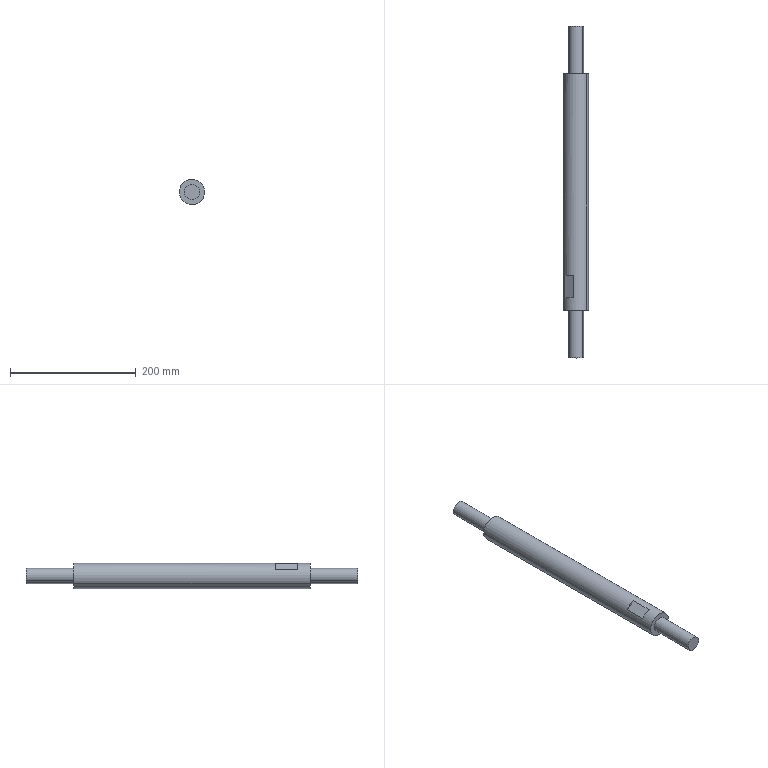Component | SolidWorks | UpperGuidePostAssembly-1_UpperSupport-1 | 1 solid | 16 faces | box 40 x 527 x 40 mm | volume 538358 mm3 | plane 10 | cylinder 6 | commonest cylinder face diameters 24 x4 40 x2
build123d program:
from build123d import *

# Parameters (mm, degrees)
CUT_EXTRUDE1_START = 30
SKETCH3_W          = 9.813
SKETCH3_H          = 35
SKETCH3_W_2        = 11.91
CUT_EXTRUDE1_DEPTH = 558.758


with BuildPart() as part:
    # Sketch1 → Revolve1 (revolve)
    with BuildSketch(Plane.XY, mode=Mode.PRIVATE) as revolve1_sk:
        Polygon((0, 527), (12, 527), (12, 451), (20, 451), (20, 76), (12, 76), (12, 0), (0, 0), align=None)
    revolve(revolve1_sk.sketch.rotate(Axis((0, 0, 0), (0, 1, 0)), 90), axis=Axis((0, 0, 0), (0, 1, 0)))

    # Sketch3 → Cut-Extrude1 (cut, through all)
    with BuildSketch(Plane.XY.offset(CUT_EXTRUDE1_START)):
        with Locations((-22.907, 413.5)):
            Rectangle(SKETCH3_W, SKETCH3_H)
        with Locations((23.955, 413.5)):
            Rectangle(SKETCH3_W_2, SKETCH3_H)
    extrude(amount=-CUT_EXTRUDE1_DEPTH, mode=Mode.SUBTRACT)


solid = part.part

# Placed as in the assembly
solid = solid.moved(Location((-407.951, 768.323, -225), (-180, -54.748, 0)))
STEP:
#1=CARTESIAN_POINT('',(-16.447,27.257,-9.131));
#2=VERTEX_POINT('',#1);
#3=CARTESIAN_POINT('',(-15.675,27.257,-8.586));
#4=VERTEX_POINT('',#3);
#5=CARTESIAN_POINT('',(-16.061,27.257,-8.858));
#6=DIRECTION('',(0.,1.,0.));
#7=DIRECTION('',(-0.8166,0.,-0.5772));
#8=AXIS2_PLACEMENT_3D('',#5,#6,#7);
#9=CIRCLE('',#8,0.4724);
#10=EDGE_CURVE('',#2,#4,#9,.T.);
#11=ORIENTED_EDGE('',*,*,#10,.T.);
#12=CARTESIAN_POINT('',(-15.675,30.249,-8.586));
#13=VERTEX_POINT('',#12);
#14=CARTESIAN_POINT('',(-15.675,30.249,-8.586));
#15=DIRECTION('',(0.,1.,0.));
#16=VECTOR('',#15,39.37);
#17=LINE('',#14,#16);
#18=EDGE_CURVE('',#4,#13,#17,.T.);
#19=ORIENTED_EDGE('',*,*,#18,.T.);
#20=CARTESIAN_POINT('',(-16.447,30.249,-9.131));
#21=VERTEX_POINT('',#20);
#22=CARTESIAN_POINT('',(-16.061,30.249,-8.858));
#23=DIRECTION('',(0.,1.,0.));
#24=DIRECTION('',(-0.8166,0.,-0.5772));
#25=AXIS2_PLACEMENT_3D('',#22,#23,#24);
#26=CIRCLE('',#25,0.4724);
#27=EDGE_CURVE('',#21,#13,#26,.T.);
#28=ORIENTED_EDGE('',*,*,#27,.F.);
#29=CARTESIAN_POINT('',(-16.447,30.249,-9.131));
#30=DIRECTION('',(0.,1.,0.));
#31=VECTOR('',#30,39.37);
#32=LINE('',#29,#31);
#33=EDGE_CURVE('',#2,#21,#32,.T.);
#34=ORIENTED_EDGE('',*,*,#33,.F.);
#35=EDGE_LOOP('',(#11,#19,#28,#34));
#36=FACE_OUTER_BOUND('',#35,.T.);
#37=CARTESIAN_POINT('',(-16.061,30.249,-8.858));
#38=DIRECTION('',(0.,1.,0.));
#39=DIRECTION('',(-0.8166,0.,-0.5772));
#40=AXIS2_PLACEMENT_3D('',#37,#38,#39);
#41=CYLINDRICAL_SURFACE('',#40,0.4724);
#42=ADVANCED_FACE('',(#36),#41,.T.);
#43=CARTESIAN_POINT('',(-16.19,14.658,-8.081));
#44=VERTEX_POINT('',#43);
#45=CARTESIAN_POINT('',(-16.75,14.658,-8.478));
#46=VERTEX_POINT('',#45);
#47=CARTESIAN_POINT('',(-16.061,14.658,-8.858));
#48=DIRECTION('',(-0.,-1.,-0.));
#49=DIRECTION('',(-0.8166,0.,-0.5772));
#50=AXIS2_PLACEMENT_3D('',#47,#48,#49);
#51=CIRCLE('',#50,0.7874);
#52=EDGE_CURVE('',#44,#46,#51,.T.);
#53=ORIENTED_EDGE('',*,*,#52,.F.);
#54=CARTESIAN_POINT('',(-16.19,13.28,-8.081));
#55=VERTEX_POINT('',#54);
#56=CARTESIAN_POINT('',(-16.19,30.249,-8.081));
#57=DIRECTION('',(0.,1.,0.));
#58=VECTOR('',#57,39.37);
#59=LINE('',#56,#58);
#60=EDGE_CURVE('',#55,#44,#59,.T.);
#61=ORIENTED_EDGE('',*,*,#60,.F.);
#62=CARTESIAN_POINT('',(-16.75,13.28,-8.478));
#63=VERTEX_POINT('',#62);
#64=CARTESIAN_POINT('',(-16.061,13.28,-8.858));
#65=DIRECTION('',(0.,1.,0.));
#66=DIRECTION('',(0.8166,0.,0.5772));
#67=AXIS2_PLACEMENT_3D('',#64,#65,#66);
#68=CIRCLE('',#67,0.7874);
#69=EDGE_CURVE('',#63,#55,#68,.T.);
#70=ORIENTED_EDGE('',*,*,#69,.F.);
#71=CARTESIAN_POINT('',(-16.75,30.249,-8.478));
#72=DIRECTION('',(-0.,-1.,-0.));
#73=VECTOR('',#72,39.37);
#74=LINE('',#71,#73);
#75=EDGE_CURVE('',#46,#63,#74,.T.);
#76=ORIENTED_EDGE('',*,*,#75,.F.);
#77=EDGE_LOOP('',(#53,#61,#70,#76));
#78=FACE_BOUND('',#77,.T.);
#79=CARTESIAN_POINT('',(-16.704,12.493,-9.313));
#80=VERTEX_POINT('',#79);
#81=CARTESIAN_POINT('',(-15.418,12.493,-8.404));
#82=VERTEX_POINT('',#81);
#83=CARTESIAN_POINT('',(-16.061,12.493,-8.858));
#84=DIRECTION('',(0.,1.,0.));
#85=DIRECTION('',(-0.8166,0.,-0.5772));
#86=AXIS2_PLACEMENT_3D('',#83,#84,#85);
#87=CIRCLE('',#86,0.7874);
#88=EDGE_CURVE('',#80,#82,#87,.T.);
#89=ORIENTED_EDGE('',*,*,#88,.T.);
#90=CARTESIAN_POINT('',(-15.418,27.257,-8.404));
#91=VERTEX_POINT('',#90);
#92=CARTESIAN_POINT('',(-15.418,30.249,-8.404));
#93=DIRECTION('',(0.,1.,0.));
#94=VECTOR('',#93,39.37);
#95=LINE('',#92,#94);
#96=EDGE_CURVE('',#82,#91,#95,.T.);
#97=ORIENTED_EDGE('',*,*,#96,.T.);
#98=CARTESIAN_POINT('',(-16.704,27.257,-9.313));
#99=VERTEX_POINT('',#98);
#100=CARTESIAN_POINT('',(-16.061,27.257,-8.858));
#101=DIRECTION('',(0.,1.,0.));
#102=DIRECTION('',(-0.8166,0.,-0.5772));
#103=AXIS2_PLACEMENT_3D('',#100,#101,#102);
#104=CIRCLE('',#103,0.7874);
#105=EDGE_CURVE('',#99,#91,#104,.T.);
#106=ORIENTED_EDGE('',*,*,#105,.F.);
#107=CARTESIAN_POINT('',(-16.704,30.249,-9.313));
#108=DIRECTION('',(0.,1.,0.));
#109=VECTOR('',#108,39.37);
#110=LINE('',#107,#109);
#111=EDGE_CURVE('',#80,#99,#110,.T.);
#112=ORIENTED_EDGE('',*,*,#111,.F.);
#113=EDGE_LOOP('',(#89,#97,#106,#112));
#114=FACE_OUTER_BOUND('',#113,.T.);
#115=CARTESIAN_POINT('',(-16.061,30.249,-8.858));
#116=DIRECTION('',(0.,1.,0.));
#117=DIRECTION('',(-0.8166,0.,-0.5772));
#118=AXIS2_PLACEMENT_3D('',#115,#116,#117);
#119=CYLINDRICAL_SURFACE('',#118,0.7874);
#120=ADVANCED_FACE('',(#78,#114),#119,.T.);
#121=CARTESIAN_POINT('',(-16.447,9.501,-9.131));
#122=VERTEX_POINT('',#121);
#123=CARTESIAN_POINT('',(-15.675,9.501,-8.586));
#124=VERTEX_POINT('',#123);
#125=CARTESIAN_POINT('',(-16.061,9.501,-8.858));
#126=DIRECTION('',(0.,1.,0.));
#127=DIRECTION('',(-0.8166,0.,-0.5772));
#128=AXIS2_PLACEMENT_3D('',#125,#126,#127);
#129=CIRCLE('',#128,0.4724);
#130=EDGE_CURVE('',#122,#124,#129,.T.);
#131=ORIENTED_EDGE('',*,*,#130,.T.);
#132=CARTESIAN_POINT('',(-15.675,12.493,-8.586));
#133=VERTEX_POINT('',#132);
#134=CARTESIAN_POINT('',(-15.675,30.249,-8.586));
#135=DIRECTION('',(0.,1.,0.));
#136=VECTOR('',#135,39.37);
#137=LINE('',#134,#136);
#138=EDGE_CURVE('',#124,#133,#137,.T.);
#139=ORIENTED_EDGE('',*,*,#138,.T.);
#140=CARTESIAN_POINT('',(-16.447,12.493,-9.131));
#141=VERTEX_POINT('',#140);
#142=CARTESIAN_POINT('',(-16.061,12.493,-8.858));
#143=DIRECTION('',(0.,1.,0.));
#144=DIRECTION('',(-0.8166,0.,-0.5772));
#145=AXIS2_PLACEMENT_3D('',#142,#143,#144);
#146=CIRCLE('',#145,0.4724);
#147=EDGE_CURVE('',#141,#133,#146,.T.);
#148=ORIENTED_EDGE('',*,*,#147,.F.);
#149=CARTESIAN_POINT('',(-16.447,30.249,-9.131));
#150=DIRECTION('',(0.,1.,0.));
#151=VECTOR('',#150,39.37);
#152=LINE('',#149,#151);
#153=EDGE_CURVE('',#122,#141,#152,.T.);
#154=ORIENTED_EDGE('',*,*,#153,.F.);
#155=EDGE_LOOP('',(#131,#139,#148,#154));
#156=FACE_OUTER_BOUND('',#155,.T.);
#157=CARTESIAN_POINT('',(-16.061,30.249,-8.858));
#158=DIRECTION('',(0.,1.,0.));
#159=DIRECTION('',(-0.8166,0.,-0.5772));
#160=AXIS2_PLACEMENT_3D('',#157,#158,#159);
#161=CYLINDRICAL_SURFACE('',#160,0.4724);
#162=ADVANCED_FACE('',(#156),#161,.T.);
#163=ORIENTED_EDGE('',*,*,#130,.F.);
#164=CARTESIAN_POINT('',(-16.061,9.501,-8.858));
#165=DIRECTION('',(0.,1.,0.));
#166=DIRECTION('',(-0.8166,0.,-0.5772));
#167=AXIS2_PLACEMENT_3D('',#164,#165,#166);
#168=CIRCLE('',#167,0.4724);
#169=EDGE_CURVE('',#124,#122,#168,.T.);
#170=ORIENTED_EDGE('',*,*,#169,.F.);
#171=EDGE_LOOP('',(#163,#170));
#172=FACE_OUTER_BOUND('',#171,.T.);
#173=CARTESIAN_POINT('',(-16.061,9.501,-8.858));
#174=DIRECTION('',(-0.,-1.,-0.));
#175=DIRECTION('',(0.8166,-0.,0.5772));
#176=AXIS2_PLACEMENT_3D('',#173,#174,#175);
#177=PLANE('',#176);
#178=ADVANCED_FACE('',(#172),#177,.T.);
#179=ORIENTED_EDGE('',*,*,#138,.F.);
#180=ORIENTED_EDGE('',*,*,#169,.T.);
#181=ORIENTED_EDGE('',*,*,#153,.T.);
#182=CARTESIAN_POINT('',(-16.061,12.493,-8.858));
#183=DIRECTION('',(0.,1.,0.));
#184=DIRECTION('',(-0.8166,0.,-0.5772));
#185=AXIS2_PLACEMENT_3D('',#182,#183,#184);
#186=CIRCLE('',#185,0.4724);
#187=EDGE_CURVE('',#133,#141,#186,.T.);
#188=ORIENTED_EDGE('',*,*,#187,.F.);
#189=EDGE_LOOP('',(#179,#180,#181,#188));
#190=FACE_OUTER_BOUND('',#189,.T.);
#191=CARTESIAN_POINT('',(-16.061,30.249,-8.858));
#192=DIRECTION('',(0.,1.,0.));
#193=DIRECTION('',(-0.8166,0.,-0.5772));
#194=AXIS2_PLACEMENT_3D('',#191,#192,#193);
#195=CYLINDRICAL_SURFACE('',#194,0.4724);
#196=ADVANCED_FACE('',(#190),#195,.T.);
#197=ORIENTED_EDGE('',*,*,#147,.T.);
#198=ORIENTED_EDGE('',*,*,#187,.T.);
#199=EDGE_LOOP('',(#197,#198));
#200=FACE_BOUND('',#199,.T.);
#201=ORIENTED_EDGE('',*,*,#88,.F.);
#202=CARTESIAN_POINT('',(-16.061,12.493,-8.858));
#203=DIRECTION('',(0.,1.,0.));
#204=DIRECTION('',(-0.8166,0.,-0.5772));
#205=AXIS2_PLACEMENT_3D('',#202,#203,#204);
#206=CIRCLE('',#205,0.7874);
#207=EDGE_CURVE('',#82,#80,#206,.T.);
#208=ORIENTED_EDGE('',*,*,#207,.F.);
#209=EDGE_LOOP('',(#201,#208));
#210=FACE_OUTER_BOUND('',#209,.T.);
#211=CARTESIAN_POINT('',(-16.334,12.493,-8.472));
#212=DIRECTION('',(-0.,-1.,-0.));
#213=DIRECTION('',(0.8166,-0.,0.5772));
#214=AXIS2_PLACEMENT_3D('',#211,#212,#213);
#215=PLANE('',#214);
#216=ADVANCED_FACE('',(#200,#210),#215,.T.);
#217=ORIENTED_EDGE('',*,*,#96,.F.);
#218=ORIENTED_EDGE('',*,*,#207,.T.);
#219=ORIENTED_EDGE('',*,*,#111,.T.);
#220=CARTESIAN_POINT('',(-16.061,27.257,-8.858));
#221=DIRECTION('',(0.,1.,0.));
#222=DIRECTION('',(-0.8166,0.,-0.5772));
#223=AXIS2_PLACEMENT_3D('',#220,#221,#222);
#224=CIRCLE('',#223,0.7874);
#225=EDGE_CURVE('',#91,#99,#224,.T.);
#226=ORIENTED_EDGE('',*,*,#225,.F.);
#227=EDGE_LOOP('',(#217,#218,#219,#226));
#228=FACE_OUTER_BOUND('',#227,.T.);
#229=CARTESIAN_POINT('',(-15.372,13.28,-9.239));
#230=VERTEX_POINT('',#229);
#231=CARTESIAN_POINT('',(-15.932,13.28,-9.635));
#232=VERTEX_POINT('',#231);
#233=CARTESIAN_POINT('',(-16.061,13.28,-8.858));
#234=DIRECTION('',(0.,1.,0.));
#235=DIRECTION('',(0.8166,0.,0.5772));
#236=AXIS2_PLACEMENT_3D('',#233,#234,#235);
#237=CIRCLE('',#236,0.7874);
#238=EDGE_CURVE('',#230,#232,#237,.T.);
#239=ORIENTED_EDGE('',*,*,#238,.F.);
#240=CARTESIAN_POINT('',(-15.372,14.658,-9.239));
#241=VERTEX_POINT('',#240);
#242=CARTESIAN_POINT('',(-15.372,30.249,-9.239));
#243=DIRECTION('',(-0.,-1.,-0.));
#244=VECTOR('',#243,39.37);
#245=LINE('',#242,#244);
#246=EDGE_CURVE('',#241,#230,#245,.T.);
#247=ORIENTED_EDGE('',*,*,#246,.F.);
#248=CARTESIAN_POINT('',(-15.932,14.658,-9.635));
#249=VERTEX_POINT('',#248);
#250=CARTESIAN_POINT('',(-16.061,14.658,-8.858));
#251=DIRECTION('',(-0.,-1.,-0.));
#252=DIRECTION('',(-0.8166,0.,-0.5772));
#253=AXIS2_PLACEMENT_3D('',#250,#251,#252);
#254=CIRCLE('',#253,0.7874);
#255=EDGE_CURVE('',#249,#241,#254,.T.);
#256=ORIENTED_EDGE('',*,*,#255,.F.);
#257=CARTESIAN_POINT('',(-15.932,30.249,-9.635));
#258=DIRECTION('',(0.,1.,0.));
#259=VECTOR('',#258,39.37);
#260=LINE('',#257,#259);
#261=EDGE_CURVE('',#232,#249,#260,.T.);
#262=ORIENTED_EDGE('',*,*,#261,.F.);
#263=EDGE_LOOP('',(#239,#247,#256,#262));
#264=FACE_BOUND('',#263,.T.);
#265=CARTESIAN_POINT('',(-16.061,30.249,-8.858));
#266=DIRECTION('',(0.,1.,0.));
#267=DIRECTION('',(-0.8166,0.,-0.5772));
#268=AXIS2_PLACEMENT_3D('',#265,#266,#267);
#269=CYLINDRICAL_SURFACE('',#268,0.7874);
#270=ADVANCED_FACE('',(#228,#264),#269,.T.);
#271=ORIENTED_EDGE('',*,*,#105,.T.);
#272=ORIENTED_EDGE('',*,*,#225,.T.);
#273=EDGE_LOOP('',(#271,#272));
#274=FACE_OUTER_BOUND('',#273,.T.);
#275=ORIENTED_EDGE('',*,*,#10,.F.);
#276=CARTESIAN_POINT('',(-16.061,27.257,-8.858));
#277=DIRECTION('',(0.,1.,0.));
#278=DIRECTION('',(-0.8166,0.,-0.5772));
#279=AXIS2_PLACEMENT_3D('',#276,#277,#278);
#280=CIRCLE('',#279,0.4724);
#281=EDGE_CURVE('',#4,#2,#280,.T.);
#282=ORIENTED_EDGE('',*,*,#281,.F.);
#283=EDGE_LOOP('',(#275,#282));
#284=FACE_BOUND('',#283,.T.);
#285=CARTESIAN_POINT('',(-16.516,27.257,-8.215));
#286=DIRECTION('',(0.,1.,0.));
#287=DIRECTION('',(-0.8166,0.,-0.5772));
#288=AXIS2_PLACEMENT_3D('',#285,#286,#287);
#289=PLANE('',#288);
#290=ADVANCED_FACE('',(#274,#284),#289,.T.);
#291=ORIENTED_EDGE('',*,*,#18,.F.);
#292=ORIENTED_EDGE('',*,*,#281,.T.);
#293=ORIENTED_EDGE('',*,*,#33,.T.);
#294=CARTESIAN_POINT('',(-16.061,30.249,-8.858));
#295=DIRECTION('',(0.,1.,0.));
#296=DIRECTION('',(-0.8166,0.,-0.5772));
#297=AXIS2_PLACEMENT_3D('',#294,#295,#296);
#298=CIRCLE('',#297,0.4724);
#299=EDGE_CURVE('',#13,#21,#298,.T.);
#300=ORIENTED_EDGE('',*,*,#299,.F.);
#301=EDGE_LOOP('',(#291,#292,#293,#300));
#302=FACE_OUTER_BOUND('',#301,.T.);
#303=CARTESIAN_POINT('',(-16.061,30.249,-8.858));
#304=DIRECTION('',(0.,1.,0.));
#305=DIRECTION('',(-0.8166,0.,-0.5772));
#306=AXIS2_PLACEMENT_3D('',#303,#304,#305);
#307=CYLINDRICAL_SURFACE('',#306,0.4724);
#308=ADVANCED_FACE('',(#302),#307,.T.);
#309=ORIENTED_EDGE('',*,*,#27,.T.);
#310=ORIENTED_EDGE('',*,*,#299,.T.);
#311=EDGE_LOOP('',(#309,#310));
#312=FACE_OUTER_BOUND('',#311,.T.);
#313=CARTESIAN_POINT('',(-16.334,30.249,-8.472));
#314=DIRECTION('',(0.,1.,0.));
#315=DIRECTION('',(-0.8166,0.,-0.5772));
#316=AXIS2_PLACEMENT_3D('',#313,#314,#315);
#317=PLANE('',#316);
#318=ADVANCED_FACE('',(#312),#317,.T.);
#319=ORIENTED_EDGE('',*,*,#238,.T.);
#320=CARTESIAN_POINT('',(-16.295,13.28,-9.891));
#321=DIRECTION('',(0.8166,-0.,0.5772));
#322=VECTOR('',#321,39.37);
#323=LINE('',#320,#322);
#324=EDGE_CURVE('',#232,#230,#323,.T.);
#325=ORIENTED_EDGE('',*,*,#324,.T.);
#326=EDGE_LOOP('',(#319,#325));
#327=FACE_OUTER_BOUND('',#326,.T.);
#328=CARTESIAN_POINT('',(-16.072,13.28,-10.207));
#329=DIRECTION('',(-0.,-1.,-0.));
#330=DIRECTION('',(0.8166,-0.,0.5772));
#331=AXIS2_PLACEMENT_3D('',#328,#329,#330);
#332=PLANE('',#331);
#333=ADVANCED_FACE('',(#327),#332,.F.);
#334=ORIENTED_EDGE('',*,*,#246,.T.);
#335=ORIENTED_EDGE('',*,*,#324,.F.);
#336=ORIENTED_EDGE('',*,*,#261,.T.);
#337=CARTESIAN_POINT('',(-16.295,14.658,-9.891));
#338=DIRECTION('',(0.8166,-0.,0.5772));
#339=VECTOR('',#338,39.37);
#340=LINE('',#337,#339);
#341=EDGE_CURVE('',#249,#241,#340,.T.);
#342=ORIENTED_EDGE('',*,*,#341,.T.);
#343=EDGE_LOOP('',(#334,#335,#336,#342));
#344=FACE_OUTER_BOUND('',#343,.T.);
#345=CARTESIAN_POINT('',(-16.295,13.28,-9.891));
#346=DIRECTION('',(-0.5772,-0.,0.8166));
#347=DIRECTION('',(-0.,-1.,-0.));
#348=AXIS2_PLACEMENT_3D('',#345,#346,#347);
#349=PLANE('',#348);
#350=ADVANCED_FACE('',(#344),#349,.F.);
#351=ORIENTED_EDGE('',*,*,#255,.T.);
#352=ORIENTED_EDGE('',*,*,#341,.F.);
#353=EDGE_LOOP('',(#351,#352));
#354=FACE_OUTER_BOUND('',#353,.T.);
#355=CARTESIAN_POINT('',(-16.072,14.658,-10.207));
#356=DIRECTION('',(0.,1.,0.));
#357=DIRECTION('',(-0.8166,0.,-0.5772));
#358=AXIS2_PLACEMENT_3D('',#355,#356,#357);
#359=PLANE('',#358);
#360=ADVANCED_FACE('',(#354),#359,.F.);
#361=ORIENTED_EDGE('',*,*,#52,.T.);
#362=CARTESIAN_POINT('',(-17.113,14.658,-8.734));
#363=DIRECTION('',(0.8166,-0.,0.5772));
#364=VECTOR('',#363,39.37);
#365=LINE('',#362,#364);
#366=EDGE_CURVE('',#46,#44,#365,.T.);
#367=ORIENTED_EDGE('',*,*,#366,.T.);
#368=EDGE_LOOP('',(#361,#367));
#369=FACE_OUTER_BOUND('',#368,.T.);
#370=CARTESIAN_POINT('',(-17.384,14.658,-8.351));
#371=DIRECTION('',(0.,1.,0.));
#372=DIRECTION('',(-0.8166,0.,-0.5772));
#373=AXIS2_PLACEMENT_3D('',#370,#371,#372);
#374=PLANE('',#373);
#375=ADVANCED_FACE('',(#369),#374,.F.);
#376=ORIENTED_EDGE('',*,*,#75,.T.);
#377=CARTESIAN_POINT('',(-17.113,13.28,-8.734));
#378=DIRECTION('',(0.8166,-0.,0.5772));
#379=VECTOR('',#378,39.37);
#380=LINE('',#377,#379);
#381=EDGE_CURVE('',#63,#55,#380,.T.);
#382=ORIENTED_EDGE('',*,*,#381,.T.);
#383=ORIENTED_EDGE('',*,*,#60,.T.);
#384=ORIENTED_EDGE('',*,*,#366,.F.);
#385=EDGE_LOOP('',(#376,#382,#383,#384));
#386=FACE_OUTER_BOUND('',#385,.T.);
#387=CARTESIAN_POINT('',(-17.113,13.28,-8.734));
#388=DIRECTION('',(0.5772,0.,-0.8166));
#389=DIRECTION('',(0.,1.,0.));
#390=AXIS2_PLACEMENT_3D('',#387,#388,#389);
#391=PLANE('',#390);
#392=ADVANCED_FACE('',(#386),#391,.F.);
#393=ORIENTED_EDGE('',*,*,#69,.T.);
#394=ORIENTED_EDGE('',*,*,#381,.F.);
#395=EDGE_LOOP('',(#393,#394));
#396=FACE_OUTER_BOUND('',#395,.T.);
#397=CARTESIAN_POINT('',(-17.384,13.28,-8.351));
#398=DIRECTION('',(-0.,-1.,-0.));
#399=DIRECTION('',(0.8166,-0.,0.5772));
#400=AXIS2_PLACEMENT_3D('',#397,#398,#399);
#401=PLANE('',#400);
#402=ADVANCED_FACE('',(#396),#401,.F.);
#403=CLOSED_SHELL('',(#42,#120,#162,#178,#196,#216,#270,#290,#308,#318,#333,#350,#360,#375,#392,#402));
#404=MANIFOLD_SOLID_BREP('',#403);
#405=CARTESIAN_POINT('',(0.,0.,0.));
#406=DIRECTION('',(0.,0.,1.));
#407=DIRECTION('',(1.,0.,0.));
#408=AXIS2_PLACEMENT_3D('',#405,#406,#407);
#409=(LENGTH_UNIT()NAMED_UNIT(*)SI_UNIT($,.METRE.));
#410=LENGTH_MEASURE_WITH_UNIT(LENGTH_MEASURE(0.0254),#409);
#411=DIMENSIONAL_EXPONENTS(1.,0.,0.,0.,0.,0.,0.);
#412=(CONVERSION_BASED_UNIT('',#410)LENGTH_UNIT()NAMED_UNIT(#411));
#413=UNCERTAINTY_MEASURE_WITH_UNIT(LENGTH_MEASURE(0.00001),#412,'','');
#414=(NAMED_UNIT(*)PLANE_ANGLE_UNIT()SI_UNIT($,.RADIAN.));
#415=(NAMED_UNIT(*)SI_UNIT($,.STERADIAN.)SOLID_ANGLE_UNIT());
#416=(GEOMETRIC_REPRESENTATION_CONTEXT(3)GLOBAL_UNCERTAINTY_ASSIGNED_CONTEXT((#413))GLOBAL_UNIT_ASSIGNED_CONTEXT((#412,#414,#415))REPRESENTATION_CONTEXT('',''));
#417=ADVANCED_BREP_SHAPE_REPRESENTATION('',(#404,#408),#416);
#418=COLOUR_RGB('',0.7922,0.8196,0.9333);
#419=FILL_AREA_STYLE_COLOUR('',#418);
#420=FILL_AREA_STYLE('',(#419));
#421=SURFACE_STYLE_FILL_AREA(#420);
#422=SURFACE_SIDE_STYLE('',(#421));
#423=SURFACE_STYLE_USAGE(.BOTH.,#422);
#424=PRESENTATION_STYLE_ASSIGNMENT((#423));
#425=STYLED_ITEM('',(#424),#404);
#426=(LENGTH_UNIT()NAMED_UNIT(*)SI_UNIT($,.METRE.));
#427=LENGTH_MEASURE_WITH_UNIT(LENGTH_MEASURE(0.0254),#426);
#428=DIMENSIONAL_EXPONENTS(1.,0.,0.,0.,0.,0.,0.);
#429=(CONVERSION_BASED_UNIT('',#427)LENGTH_UNIT()NAMED_UNIT(#428));
#430=UNCERTAINTY_MEASURE_WITH_UNIT(LENGTH_MEASURE(0.00001),#429,'','');
#431=(NAMED_UNIT(*)PLANE_ANGLE_UNIT()SI_UNIT($,.RADIAN.));
#432=(NAMED_UNIT(*)SI_UNIT($,.STERADIAN.)SOLID_ANGLE_UNIT());
#433=(GEOMETRIC_REPRESENTATION_CONTEXT(3)GLOBAL_UNCERTAINTY_ASSIGNED_CONTEXT((#430))GLOBAL_UNIT_ASSIGNED_CONTEXT((#429,#431,#432))REPRESENTATION_CONTEXT('',''));
#434=MECHANICAL_DESIGN_GEOMETRIC_PRESENTATION_REPRESENTATION('',(#425),#433);
#435=PRESENTATION_LAYER_ASSIGNMENT('','',(#425));